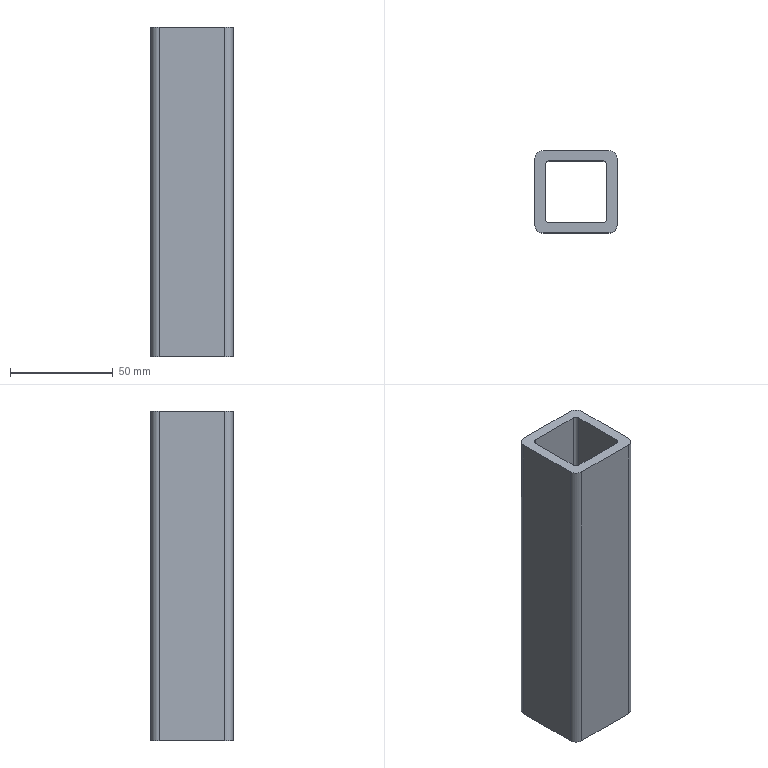Component | SolidWorks | 40-40SquareTube8-2 | 1 solid | 18 faces | box 40 x 40 x 160 mm | volume 110352 mm3 | plane 10 | cylinder 8 | commonest cylinder face diameters 8 x4 4 x4
build123d program:
from build123d import *

# Parameters (mm, degrees)
BOSS_EXTRUDE1_DEPTH = 80


with BuildPart() as part:
    # Sketch1 → Boss-Extrude1 (new, symmetric)
    with BuildSketch(Plane.XY):
        with BuildLine():
            Line((-16, -20), (16, -20))
            ThreePointArc((16, -20), (18.828, -18.828), (20, -16))
            Line((20, -16), (20, 16))
            ThreePointArc((20, 16), (18.828, 18.828), (16, 20))
            Line((16, 20), (-16, 20))
            ThreePointArc((-16, 20), (-18.828, 18.828), (-20, 16))
            Line((-20, 16), (-20, -16))
            ThreePointArc((-20, -16), (-18.828, -18.828), (-16, -20))
        make_face()
        with BuildLine():
            Line((-13, -15), (13, -15))
            ThreePointArc((13, -15), (14.414, -14.414), (15, -13))
            Line((15, -13), (15, 13))
            ThreePointArc((15, 13), (14.414, 14.414), (13, 15))
            Line((13, 15), (-13, 15))
            ThreePointArc((-13, 15), (-14.414, 14.414), (-15, 13))
            Line((-15, 13), (-15, -13))
            ThreePointArc((-15, -13), (-14.414, -14.414), (-13, -15))
        make_face(mode=Mode.SUBTRACT)
    extrude(amount=BOSS_EXTRUDE1_DEPTH, both=True)


solid = part.part

# Placed as in the assembly
solid = solid.moved(Location((17.398, 447.837, 100), (0, 0, 0)))
STEP:
#1=CARTESIAN_POINT('',(1.315,16.844,7.087));
#2=VERTEX_POINT('',#1);
#3=CARTESIAN_POINT('',(1.472,17.001,7.087));
#4=VERTEX_POINT('',#3);
#5=CARTESIAN_POINT('',(1.315,17.001,7.087));
#6=DIRECTION('',(0.,0.,1.));
#7=DIRECTION('',(1.,0.,0.));
#8=AXIS2_PLACEMENT_3D('',#5,#6,#7);
#9=CIRCLE('',#8,0.1575);
#10=EDGE_CURVE('',#2,#4,#9,.T.);
#11=ORIENTED_EDGE('',*,*,#10,.T.);
#12=CARTESIAN_POINT('',(1.472,18.261,7.087));
#13=VERTEX_POINT('',#12);
#14=CARTESIAN_POINT('',(1.472,17.001,7.087));
#15=DIRECTION('',(0.,1.,0.));
#16=VECTOR('',#15,39.37);
#17=LINE('',#14,#16);
#18=EDGE_CURVE('',#4,#13,#17,.T.);
#19=ORIENTED_EDGE('',*,*,#18,.T.);
#20=CARTESIAN_POINT('',(1.315,18.419,7.087));
#21=VERTEX_POINT('',#20);
#22=CARTESIAN_POINT('',(1.315,18.261,7.087));
#23=DIRECTION('',(0.,0.,1.));
#24=DIRECTION('',(-1.,0.,0.));
#25=AXIS2_PLACEMENT_3D('',#22,#23,#24);
#26=CIRCLE('',#25,0.1575);
#27=EDGE_CURVE('',#13,#21,#26,.T.);
#28=ORIENTED_EDGE('',*,*,#27,.T.);
#29=CARTESIAN_POINT('',(0.05504,18.419,7.087));
#30=VERTEX_POINT('',#29);
#31=CARTESIAN_POINT('',(0.05504,18.419,7.087));
#32=DIRECTION('',(-1.,0.,0.));
#33=VECTOR('',#32,39.37);
#34=LINE('',#31,#33);
#35=EDGE_CURVE('',#21,#30,#34,.T.);
#36=ORIENTED_EDGE('',*,*,#35,.T.);
#37=CARTESIAN_POINT('',(-0.1024,18.261,7.087));
#38=VERTEX_POINT('',#37);
#39=CARTESIAN_POINT('',(0.05504,18.261,7.087));
#40=DIRECTION('',(0.,0.,1.));
#41=DIRECTION('',(-1.,0.,0.));
#42=AXIS2_PLACEMENT_3D('',#39,#40,#41);
#43=CIRCLE('',#42,0.1575);
#44=EDGE_CURVE('',#30,#38,#43,.T.);
#45=ORIENTED_EDGE('',*,*,#44,.T.);
#46=CARTESIAN_POINT('',(-0.1024,17.001,7.087));
#47=VERTEX_POINT('',#46);
#48=CARTESIAN_POINT('',(-0.1024,17.001,7.087));
#49=DIRECTION('',(-0.,-1.,0.));
#50=VECTOR('',#49,39.37);
#51=LINE('',#48,#50);
#52=EDGE_CURVE('',#38,#47,#51,.T.);
#53=ORIENTED_EDGE('',*,*,#52,.T.);
#54=CARTESIAN_POINT('',(0.05504,16.844,7.087));
#55=VERTEX_POINT('',#54);
#56=CARTESIAN_POINT('',(0.05504,17.001,7.087));
#57=DIRECTION('',(0.,0.,1.));
#58=DIRECTION('',(-1.,0.,0.));
#59=AXIS2_PLACEMENT_3D('',#56,#57,#58);
#60=CIRCLE('',#59,0.1575);
#61=EDGE_CURVE('',#47,#55,#60,.T.);
#62=ORIENTED_EDGE('',*,*,#61,.T.);
#63=CARTESIAN_POINT('',(0.05504,16.844,7.087));
#64=DIRECTION('',(1.,0.,0.));
#65=VECTOR('',#64,39.37);
#66=LINE('',#63,#65);
#67=EDGE_CURVE('',#55,#2,#66,.T.);
#68=ORIENTED_EDGE('',*,*,#67,.T.);
#69=EDGE_LOOP('',(#11,#19,#28,#36,#45,#53,#62,#68));
#70=FACE_OUTER_BOUND('',#69,.T.);
#71=CARTESIAN_POINT('',(1.276,17.12,7.087));
#72=VERTEX_POINT('',#71);
#73=CARTESIAN_POINT('',(1.276,18.143,7.087));
#74=VERTEX_POINT('',#73);
#75=CARTESIAN_POINT('',(1.276,17.12,7.087));
#76=DIRECTION('',(0.,1.,0.));
#77=VECTOR('',#76,39.37);
#78=LINE('',#75,#77);
#79=EDGE_CURVE('',#72,#74,#78,.T.);
#80=ORIENTED_EDGE('',*,*,#79,.F.);
#81=CARTESIAN_POINT('',(1.197,17.041,7.087));
#82=VERTEX_POINT('',#81);
#83=CARTESIAN_POINT('',(1.197,17.12,7.087));
#84=DIRECTION('',(0.,0.,1.));
#85=DIRECTION('',(1.,0.,0.));
#86=AXIS2_PLACEMENT_3D('',#83,#84,#85);
#87=CIRCLE('',#86,0.07874);
#88=EDGE_CURVE('',#82,#72,#87,.T.);
#89=ORIENTED_EDGE('',*,*,#88,.F.);
#90=CARTESIAN_POINT('',(0.1732,17.041,7.087));
#91=VERTEX_POINT('',#90);
#92=CARTESIAN_POINT('',(0.1732,17.041,7.087));
#93=DIRECTION('',(1.,0.,0.));
#94=VECTOR('',#93,39.37);
#95=LINE('',#92,#94);
#96=EDGE_CURVE('',#91,#82,#95,.T.);
#97=ORIENTED_EDGE('',*,*,#96,.F.);
#98=CARTESIAN_POINT('',(0.09441,17.12,7.087));
#99=VERTEX_POINT('',#98);
#100=CARTESIAN_POINT('',(0.1732,17.12,7.087));
#101=DIRECTION('',(0.,0.,1.));
#102=DIRECTION('',(-1.,0.,0.));
#103=AXIS2_PLACEMENT_3D('',#100,#101,#102);
#104=CIRCLE('',#103,0.07874);
#105=EDGE_CURVE('',#99,#91,#104,.T.);
#106=ORIENTED_EDGE('',*,*,#105,.F.);
#107=CARTESIAN_POINT('',(0.09441,18.143,7.087));
#108=VERTEX_POINT('',#107);
#109=CARTESIAN_POINT('',(0.09441,17.12,7.087));
#110=DIRECTION('',(0.,-1.,0.));
#111=VECTOR('',#110,39.37);
#112=LINE('',#109,#111);
#113=EDGE_CURVE('',#108,#99,#112,.T.);
#114=ORIENTED_EDGE('',*,*,#113,.F.);
#115=CARTESIAN_POINT('',(0.1732,18.222,7.087));
#116=VERTEX_POINT('',#115);
#117=CARTESIAN_POINT('',(0.1732,18.143,7.087));
#118=DIRECTION('',(0.,0.,1.));
#119=DIRECTION('',(-1.,0.,0.));
#120=AXIS2_PLACEMENT_3D('',#117,#118,#119);
#121=CIRCLE('',#120,0.07874);
#122=EDGE_CURVE('',#116,#108,#121,.T.);
#123=ORIENTED_EDGE('',*,*,#122,.F.);
#124=CARTESIAN_POINT('',(1.197,18.222,7.087));
#125=VERTEX_POINT('',#124);
#126=CARTESIAN_POINT('',(0.1732,18.222,7.087));
#127=DIRECTION('',(-1.,0.,0.));
#128=VECTOR('',#127,39.37);
#129=LINE('',#126,#128);
#130=EDGE_CURVE('',#125,#116,#129,.T.);
#131=ORIENTED_EDGE('',*,*,#130,.F.);
#132=CARTESIAN_POINT('',(1.197,18.143,7.087));
#133=DIRECTION('',(0.,0.,1.));
#134=DIRECTION('',(-1.,0.,0.));
#135=AXIS2_PLACEMENT_3D('',#132,#133,#134);
#136=CIRCLE('',#135,0.07874);
#137=EDGE_CURVE('',#74,#125,#136,.T.);
#138=ORIENTED_EDGE('',*,*,#137,.F.);
#139=EDGE_LOOP('',(#80,#89,#97,#106,#114,#123,#131,#138));
#140=FACE_BOUND('',#139,.T.);
#141=CARTESIAN_POINT('',(1.315,17.001,7.087));
#142=DIRECTION('',(0.,0.,1.));
#143=DIRECTION('',(1.,0.,0.));
#144=AXIS2_PLACEMENT_3D('',#141,#142,#143);
#145=PLANE('',#144);
#146=ADVANCED_FACE('',(#70,#140),#145,.T.);
#147=CARTESIAN_POINT('',(1.315,16.844,0.7874));
#148=VERTEX_POINT('',#147);
#149=CARTESIAN_POINT('',(1.472,17.001,0.7874));
#150=VERTEX_POINT('',#149);
#151=CARTESIAN_POINT('',(1.315,17.001,0.7874));
#152=DIRECTION('',(0.,0.,1.));
#153=DIRECTION('',(1.,0.,0.));
#154=AXIS2_PLACEMENT_3D('',#151,#152,#153);
#155=CIRCLE('',#154,0.1575);
#156=EDGE_CURVE('',#148,#150,#155,.T.);
#157=ORIENTED_EDGE('',*,*,#156,.F.);
#158=CARTESIAN_POINT('',(0.05504,16.844,0.7874));
#159=VERTEX_POINT('',#158);
#160=CARTESIAN_POINT('',(0.05504,16.844,0.7874));
#161=DIRECTION('',(1.,0.,0.));
#162=VECTOR('',#161,39.37);
#163=LINE('',#160,#162);
#164=EDGE_CURVE('',#159,#148,#163,.T.);
#165=ORIENTED_EDGE('',*,*,#164,.F.);
#166=CARTESIAN_POINT('',(-0.1024,17.001,0.7874));
#167=VERTEX_POINT('',#166);
#168=CARTESIAN_POINT('',(0.05504,17.001,0.7874));
#169=DIRECTION('',(0.,0.,1.));
#170=DIRECTION('',(-1.,0.,0.));
#171=AXIS2_PLACEMENT_3D('',#168,#169,#170);
#172=CIRCLE('',#171,0.1575);
#173=EDGE_CURVE('',#167,#159,#172,.T.);
#174=ORIENTED_EDGE('',*,*,#173,.F.);
#175=CARTESIAN_POINT('',(-0.1024,18.261,0.7874));
#176=VERTEX_POINT('',#175);
#177=CARTESIAN_POINT('',(-0.1024,17.001,0.7874));
#178=DIRECTION('',(-0.,-1.,0.));
#179=VECTOR('',#178,39.37);
#180=LINE('',#177,#179);
#181=EDGE_CURVE('',#176,#167,#180,.T.);
#182=ORIENTED_EDGE('',*,*,#181,.F.);
#183=CARTESIAN_POINT('',(0.05504,18.419,0.7874));
#184=VERTEX_POINT('',#183);
#185=CARTESIAN_POINT('',(0.05504,18.261,0.7874));
#186=DIRECTION('',(0.,0.,1.));
#187=DIRECTION('',(-1.,0.,0.));
#188=AXIS2_PLACEMENT_3D('',#185,#186,#187);
#189=CIRCLE('',#188,0.1575);
#190=EDGE_CURVE('',#184,#176,#189,.T.);
#191=ORIENTED_EDGE('',*,*,#190,.F.);
#192=CARTESIAN_POINT('',(1.315,18.419,0.7874));
#193=VERTEX_POINT('',#192);
#194=CARTESIAN_POINT('',(0.05504,18.419,0.7874));
#195=DIRECTION('',(-1.,0.,0.));
#196=VECTOR('',#195,39.37);
#197=LINE('',#194,#196);
#198=EDGE_CURVE('',#193,#184,#197,.T.);
#199=ORIENTED_EDGE('',*,*,#198,.F.);
#200=CARTESIAN_POINT('',(1.472,18.261,0.7874));
#201=VERTEX_POINT('',#200);
#202=CARTESIAN_POINT('',(1.315,18.261,0.7874));
#203=DIRECTION('',(0.,0.,1.));
#204=DIRECTION('',(-1.,0.,0.));
#205=AXIS2_PLACEMENT_3D('',#202,#203,#204);
#206=CIRCLE('',#205,0.1575);
#207=EDGE_CURVE('',#201,#193,#206,.T.);
#208=ORIENTED_EDGE('',*,*,#207,.F.);
#209=CARTESIAN_POINT('',(1.472,17.001,0.7874));
#210=DIRECTION('',(0.,1.,0.));
#211=VECTOR('',#210,39.37);
#212=LINE('',#209,#211);
#213=EDGE_CURVE('',#150,#201,#212,.T.);
#214=ORIENTED_EDGE('',*,*,#213,.F.);
#215=EDGE_LOOP('',(#157,#165,#174,#182,#191,#199,#208,#214));
#216=FACE_OUTER_BOUND('',#215,.T.);
#217=CARTESIAN_POINT('',(1.197,17.041,0.7874));
#218=VERTEX_POINT('',#217);
#219=CARTESIAN_POINT('',(1.276,17.12,0.7874));
#220=VERTEX_POINT('',#219);
#221=CARTESIAN_POINT('',(1.197,17.12,0.7874));
#222=DIRECTION('',(0.,0.,1.));
#223=DIRECTION('',(1.,0.,0.));
#224=AXIS2_PLACEMENT_3D('',#221,#222,#223);
#225=CIRCLE('',#224,0.07874);
#226=EDGE_CURVE('',#218,#220,#225,.T.);
#227=ORIENTED_EDGE('',*,*,#226,.T.);
#228=CARTESIAN_POINT('',(1.276,18.143,0.7874));
#229=VERTEX_POINT('',#228);
#230=CARTESIAN_POINT('',(1.276,17.12,0.7874));
#231=DIRECTION('',(0.,1.,0.));
#232=VECTOR('',#231,39.37);
#233=LINE('',#230,#232);
#234=EDGE_CURVE('',#220,#229,#233,.T.);
#235=ORIENTED_EDGE('',*,*,#234,.T.);
#236=CARTESIAN_POINT('',(1.197,18.222,0.7874));
#237=VERTEX_POINT('',#236);
#238=CARTESIAN_POINT('',(1.197,18.143,0.7874));
#239=DIRECTION('',(0.,0.,1.));
#240=DIRECTION('',(-1.,0.,0.));
#241=AXIS2_PLACEMENT_3D('',#238,#239,#240);
#242=CIRCLE('',#241,0.07874);
#243=EDGE_CURVE('',#229,#237,#242,.T.);
#244=ORIENTED_EDGE('',*,*,#243,.T.);
#245=CARTESIAN_POINT('',(0.1732,18.222,0.7874));
#246=VERTEX_POINT('',#245);
#247=CARTESIAN_POINT('',(0.1732,18.222,0.7874));
#248=DIRECTION('',(-1.,0.,0.));
#249=VECTOR('',#248,39.37);
#250=LINE('',#247,#249);
#251=EDGE_CURVE('',#237,#246,#250,.T.);
#252=ORIENTED_EDGE('',*,*,#251,.T.);
#253=CARTESIAN_POINT('',(0.09441,18.143,0.7874));
#254=VERTEX_POINT('',#253);
#255=CARTESIAN_POINT('',(0.1732,18.143,0.7874));
#256=DIRECTION('',(0.,0.,1.));
#257=DIRECTION('',(-1.,0.,0.));
#258=AXIS2_PLACEMENT_3D('',#255,#256,#257);
#259=CIRCLE('',#258,0.07874);
#260=EDGE_CURVE('',#246,#254,#259,.T.);
#261=ORIENTED_EDGE('',*,*,#260,.T.);
#262=CARTESIAN_POINT('',(0.09441,17.12,0.7874));
#263=VERTEX_POINT('',#262);
#264=CARTESIAN_POINT('',(0.09441,17.12,0.7874));
#265=DIRECTION('',(0.,-1.,0.));
#266=VECTOR('',#265,39.37);
#267=LINE('',#264,#266);
#268=EDGE_CURVE('',#254,#263,#267,.T.);
#269=ORIENTED_EDGE('',*,*,#268,.T.);
#270=CARTESIAN_POINT('',(0.1732,17.041,0.7874));
#271=VERTEX_POINT('',#270);
#272=CARTESIAN_POINT('',(0.1732,17.12,0.7874));
#273=DIRECTION('',(0.,0.,1.));
#274=DIRECTION('',(-1.,0.,0.));
#275=AXIS2_PLACEMENT_3D('',#272,#273,#274);
#276=CIRCLE('',#275,0.07874);
#277=EDGE_CURVE('',#263,#271,#276,.T.);
#278=ORIENTED_EDGE('',*,*,#277,.T.);
#279=CARTESIAN_POINT('',(0.1732,17.041,0.7874));
#280=DIRECTION('',(1.,0.,0.));
#281=VECTOR('',#280,39.37);
#282=LINE('',#279,#281);
#283=EDGE_CURVE('',#271,#218,#282,.T.);
#284=ORIENTED_EDGE('',*,*,#283,.T.);
#285=EDGE_LOOP('',(#227,#235,#244,#252,#261,#269,#278,#284));
#286=FACE_BOUND('',#285,.T.);
#287=CARTESIAN_POINT('',(1.315,17.001,0.7874));
#288=DIRECTION('',(0.,0.,1.));
#289=DIRECTION('',(1.,0.,0.));
#290=AXIS2_PLACEMENT_3D('',#287,#288,#289);
#291=PLANE('',#290);
#292=ADVANCED_FACE('',(#216,#286),#291,.F.);
#293=ORIENTED_EDGE('',*,*,#156,.T.);
#294=CARTESIAN_POINT('',(1.472,17.001,7.087));
#295=DIRECTION('',(0.,0.,-1.));
#296=VECTOR('',#295,39.37);
#297=LINE('',#294,#296);
#298=EDGE_CURVE('',#4,#150,#297,.T.);
#299=ORIENTED_EDGE('',*,*,#298,.F.);
#300=ORIENTED_EDGE('',*,*,#10,.F.);
#301=CARTESIAN_POINT('',(1.315,16.844,7.087));
#302=DIRECTION('',(0.,0.,-1.));
#303=VECTOR('',#302,39.37);
#304=LINE('',#301,#303);
#305=EDGE_CURVE('',#2,#148,#304,.T.);
#306=ORIENTED_EDGE('',*,*,#305,.T.);
#307=EDGE_LOOP('',(#293,#299,#300,#306));
#308=FACE_OUTER_BOUND('',#307,.T.);
#309=CARTESIAN_POINT('',(1.315,17.001,7.087));
#310=DIRECTION('',(0.,0.,-1.));
#311=DIRECTION('',(-1.,0.,0.));
#312=AXIS2_PLACEMENT_3D('',#309,#310,#311);
#313=CYLINDRICAL_SURFACE('',#312,0.1575);
#314=ADVANCED_FACE('',(#308),#313,.T.);
#315=ORIENTED_EDGE('',*,*,#213,.T.);
#316=CARTESIAN_POINT('',(1.472,18.261,7.087));
#317=DIRECTION('',(0.,0.,-1.));
#318=VECTOR('',#317,39.37);
#319=LINE('',#316,#318);
#320=EDGE_CURVE('',#13,#201,#319,.T.);
#321=ORIENTED_EDGE('',*,*,#320,.F.);
#322=ORIENTED_EDGE('',*,*,#18,.F.);
#323=ORIENTED_EDGE('',*,*,#298,.T.);
#324=EDGE_LOOP('',(#315,#321,#322,#323));
#325=FACE_OUTER_BOUND('',#324,.T.);
#326=CARTESIAN_POINT('',(1.472,17.001,7.087));
#327=DIRECTION('',(-1.,0.,0.));
#328=DIRECTION('',(0.,0.,1.));
#329=AXIS2_PLACEMENT_3D('',#326,#327,#328);
#330=PLANE('',#329);
#331=ADVANCED_FACE('',(#325),#330,.F.);
#332=ORIENTED_EDGE('',*,*,#207,.T.);
#333=CARTESIAN_POINT('',(1.315,18.419,7.087));
#334=DIRECTION('',(0.,0.,-1.));
#335=VECTOR('',#334,39.37);
#336=LINE('',#333,#335);
#337=EDGE_CURVE('',#21,#193,#336,.T.);
#338=ORIENTED_EDGE('',*,*,#337,.F.);
#339=ORIENTED_EDGE('',*,*,#27,.F.);
#340=ORIENTED_EDGE('',*,*,#320,.T.);
#341=EDGE_LOOP('',(#332,#338,#339,#340));
#342=FACE_OUTER_BOUND('',#341,.T.);
#343=CARTESIAN_POINT('',(1.315,18.261,7.087));
#344=DIRECTION('',(0.,0.,-1.));
#345=DIRECTION('',(-1.,0.,0.));
#346=AXIS2_PLACEMENT_3D('',#343,#344,#345);
#347=CYLINDRICAL_SURFACE('',#346,0.1575);
#348=ADVANCED_FACE('',(#342),#347,.T.);
#349=ORIENTED_EDGE('',*,*,#198,.T.);
#350=CARTESIAN_POINT('',(0.05504,18.419,7.087));
#351=DIRECTION('',(0.,0.,-1.));
#352=VECTOR('',#351,39.37);
#353=LINE('',#350,#352);
#354=EDGE_CURVE('',#30,#184,#353,.T.);
#355=ORIENTED_EDGE('',*,*,#354,.F.);
#356=ORIENTED_EDGE('',*,*,#35,.F.);
#357=ORIENTED_EDGE('',*,*,#337,.T.);
#358=EDGE_LOOP('',(#349,#355,#356,#357));
#359=FACE_OUTER_BOUND('',#358,.T.);
#360=CARTESIAN_POINT('',(0.05504,18.419,7.087));
#361=DIRECTION('',(0.,-1.,0.));
#362=DIRECTION('',(0.,0.,-1.));
#363=AXIS2_PLACEMENT_3D('',#360,#361,#362);
#364=PLANE('',#363);
#365=ADVANCED_FACE('',(#359),#364,.F.);
#366=ORIENTED_EDGE('',*,*,#190,.T.);
#367=CARTESIAN_POINT('',(-0.1024,18.261,7.087));
#368=DIRECTION('',(0.,0.,-1.));
#369=VECTOR('',#368,39.37);
#370=LINE('',#367,#369);
#371=EDGE_CURVE('',#38,#176,#370,.T.);
#372=ORIENTED_EDGE('',*,*,#371,.F.);
#373=ORIENTED_EDGE('',*,*,#44,.F.);
#374=ORIENTED_EDGE('',*,*,#354,.T.);
#375=EDGE_LOOP('',(#366,#372,#373,#374));
#376=FACE_OUTER_BOUND('',#375,.T.);
#377=CARTESIAN_POINT('',(0.05504,18.261,7.087));
#378=DIRECTION('',(0.,0.,-1.));
#379=DIRECTION('',(-1.,0.,0.));
#380=AXIS2_PLACEMENT_3D('',#377,#378,#379);
#381=CYLINDRICAL_SURFACE('',#380,0.1575);
#382=ADVANCED_FACE('',(#376),#381,.T.);
#383=ORIENTED_EDGE('',*,*,#181,.T.);
#384=CARTESIAN_POINT('',(-0.1024,17.001,7.087));
#385=DIRECTION('',(0.,0.,-1.));
#386=VECTOR('',#385,39.37);
#387=LINE('',#384,#386);
#388=EDGE_CURVE('',#47,#167,#387,.T.);
#389=ORIENTED_EDGE('',*,*,#388,.F.);
#390=ORIENTED_EDGE('',*,*,#52,.F.);
#391=ORIENTED_EDGE('',*,*,#371,.T.);
#392=EDGE_LOOP('',(#383,#389,#390,#391));
#393=FACE_OUTER_BOUND('',#392,.T.);
#394=CARTESIAN_POINT('',(-0.1024,17.001,7.087));
#395=DIRECTION('',(1.,-0.,0.));
#396=DIRECTION('',(0.,1.,0.));
#397=AXIS2_PLACEMENT_3D('',#394,#395,#396);
#398=PLANE('',#397);
#399=ADVANCED_FACE('',(#393),#398,.F.);
#400=ORIENTED_EDGE('',*,*,#173,.T.);
#401=CARTESIAN_POINT('',(0.05504,16.844,7.087));
#402=DIRECTION('',(0.,0.,-1.));
#403=VECTOR('',#402,39.37);
#404=LINE('',#401,#403);
#405=EDGE_CURVE('',#55,#159,#404,.T.);
#406=ORIENTED_EDGE('',*,*,#405,.F.);
#407=ORIENTED_EDGE('',*,*,#61,.F.);
#408=ORIENTED_EDGE('',*,*,#388,.T.);
#409=EDGE_LOOP('',(#400,#406,#407,#408));
#410=FACE_OUTER_BOUND('',#409,.T.);
#411=CARTESIAN_POINT('',(0.05504,17.001,7.087));
#412=DIRECTION('',(0.,0.,-1.));
#413=DIRECTION('',(-1.,0.,0.));
#414=AXIS2_PLACEMENT_3D('',#411,#412,#413);
#415=CYLINDRICAL_SURFACE('',#414,0.1575);
#416=ADVANCED_FACE('',(#410),#415,.T.);
#417=ORIENTED_EDGE('',*,*,#164,.T.);
#418=ORIENTED_EDGE('',*,*,#305,.F.);
#419=ORIENTED_EDGE('',*,*,#67,.F.);
#420=ORIENTED_EDGE('',*,*,#405,.T.);
#421=EDGE_LOOP('',(#417,#418,#419,#420));
#422=FACE_OUTER_BOUND('',#421,.T.);
#423=CARTESIAN_POINT('',(0.05504,16.844,7.087));
#424=DIRECTION('',(0.,1.,0.));
#425=DIRECTION('',(0.,0.,1.));
#426=AXIS2_PLACEMENT_3D('',#423,#424,#425);
#427=PLANE('',#426);
#428=ADVANCED_FACE('',(#422),#427,.F.);
#429=ORIENTED_EDGE('',*,*,#226,.F.);
#430=CARTESIAN_POINT('',(1.197,17.041,7.087));
#431=DIRECTION('',(0.,0.,-1.));
#432=VECTOR('',#431,39.37);
#433=LINE('',#430,#432);
#434=EDGE_CURVE('',#82,#218,#433,.T.);
#435=ORIENTED_EDGE('',*,*,#434,.F.);
#436=ORIENTED_EDGE('',*,*,#88,.T.);
#437=CARTESIAN_POINT('',(1.276,17.12,7.087));
#438=DIRECTION('',(0.,0.,-1.));
#439=VECTOR('',#438,39.37);
#440=LINE('',#437,#439);
#441=EDGE_CURVE('',#72,#220,#440,.T.);
#442=ORIENTED_EDGE('',*,*,#441,.T.);
#443=EDGE_LOOP('',(#429,#435,#436,#442));
#444=FACE_OUTER_BOUND('',#443,.T.);
#445=CARTESIAN_POINT('',(1.197,17.12,7.087));
#446=DIRECTION('',(0.,0.,-1.));
#447=DIRECTION('',(-1.,0.,0.));
#448=AXIS2_PLACEMENT_3D('',#445,#446,#447);
#449=CYLINDRICAL_SURFACE('',#448,0.07874);
#450=ADVANCED_FACE('',(#444),#449,.F.);
#451=ORIENTED_EDGE('',*,*,#234,.F.);
#452=ORIENTED_EDGE('',*,*,#441,.F.);
#453=ORIENTED_EDGE('',*,*,#79,.T.);
#454=CARTESIAN_POINT('',(1.276,18.143,7.087));
#455=DIRECTION('',(0.,0.,-1.));
#456=VECTOR('',#455,39.37);
#457=LINE('',#454,#456);
#458=EDGE_CURVE('',#74,#229,#457,.T.);
#459=ORIENTED_EDGE('',*,*,#458,.T.);
#460=EDGE_LOOP('',(#451,#452,#453,#459));
#461=FACE_OUTER_BOUND('',#460,.T.);
#462=CARTESIAN_POINT('',(1.276,17.12,7.087));
#463=DIRECTION('',(-1.,0.,0.));
#464=DIRECTION('',(0.,0.,1.));
#465=AXIS2_PLACEMENT_3D('',#462,#463,#464);
#466=PLANE('',#465);
#467=ADVANCED_FACE('',(#461),#466,.T.);
#468=ORIENTED_EDGE('',*,*,#243,.F.);
#469=ORIENTED_EDGE('',*,*,#458,.F.);
#470=ORIENTED_EDGE('',*,*,#137,.T.);
#471=CARTESIAN_POINT('',(1.197,18.222,7.087));
#472=DIRECTION('',(0.,0.,-1.));
#473=VECTOR('',#472,39.37);
#474=LINE('',#471,#473);
#475=EDGE_CURVE('',#125,#237,#474,.T.);
#476=ORIENTED_EDGE('',*,*,#475,.T.);
#477=EDGE_LOOP('',(#468,#469,#470,#476));
#478=FACE_OUTER_BOUND('',#477,.T.);
#479=CARTESIAN_POINT('',(1.197,18.143,7.087));
#480=DIRECTION('',(0.,0.,-1.));
#481=DIRECTION('',(-1.,0.,0.));
#482=AXIS2_PLACEMENT_3D('',#479,#480,#481);
#483=CYLINDRICAL_SURFACE('',#482,0.07874);
#484=ADVANCED_FACE('',(#478),#483,.F.);
#485=ORIENTED_EDGE('',*,*,#251,.F.);
#486=ORIENTED_EDGE('',*,*,#475,.F.);
#487=ORIENTED_EDGE('',*,*,#130,.T.);
#488=CARTESIAN_POINT('',(0.1732,18.222,7.087));
#489=DIRECTION('',(0.,0.,-1.));
#490=VECTOR('',#489,39.37);
#491=LINE('',#488,#490);
#492=EDGE_CURVE('',#116,#246,#491,.T.);
#493=ORIENTED_EDGE('',*,*,#492,.T.);
#494=EDGE_LOOP('',(#485,#486,#487,#493));
#495=FACE_OUTER_BOUND('',#494,.T.);
#496=CARTESIAN_POINT('',(0.1732,18.222,7.087));
#497=DIRECTION('',(0.,-1.,0.));
#498=DIRECTION('',(0.,0.,-1.));
#499=AXIS2_PLACEMENT_3D('',#496,#497,#498);
#500=PLANE('',#499);
#501=ADVANCED_FACE('',(#495),#500,.T.);
#502=ORIENTED_EDGE('',*,*,#260,.F.);
#503=ORIENTED_EDGE('',*,*,#492,.F.);
#504=ORIENTED_EDGE('',*,*,#122,.T.);
#505=CARTESIAN_POINT('',(0.09441,18.143,7.087));
#506=DIRECTION('',(0.,0.,-1.));
#507=VECTOR('',#506,39.37);
#508=LINE('',#505,#507);
#509=EDGE_CURVE('',#108,#254,#508,.T.);
#510=ORIENTED_EDGE('',*,*,#509,.T.);
#511=EDGE_LOOP('',(#502,#503,#504,#510));
#512=FACE_OUTER_BOUND('',#511,.T.);
#513=CARTESIAN_POINT('',(0.1732,18.143,7.087));
#514=DIRECTION('',(0.,0.,-1.));
#515=DIRECTION('',(-1.,0.,0.));
#516=AXIS2_PLACEMENT_3D('',#513,#514,#515);
#517=CYLINDRICAL_SURFACE('',#516,0.07874);
#518=ADVANCED_FACE('',(#512),#517,.F.);
#519=ORIENTED_EDGE('',*,*,#268,.F.);
#520=ORIENTED_EDGE('',*,*,#509,.F.);
#521=ORIENTED_EDGE('',*,*,#113,.T.);
#522=CARTESIAN_POINT('',(0.09441,17.12,7.087));
#523=DIRECTION('',(0.,0.,-1.));
#524=VECTOR('',#523,39.37);
#525=LINE('',#522,#524);
#526=EDGE_CURVE('',#99,#263,#525,.T.);
#527=ORIENTED_EDGE('',*,*,#526,.T.);
#528=EDGE_LOOP('',(#519,#520,#521,#527));
#529=FACE_OUTER_BOUND('',#528,.T.);
#530=CARTESIAN_POINT('',(0.09441,17.12,7.087));
#531=DIRECTION('',(1.,0.,0.));
#532=DIRECTION('',(0.,0.,-1.));
#533=AXIS2_PLACEMENT_3D('',#530,#531,#532);
#534=PLANE('',#533);
#535=ADVANCED_FACE('',(#529),#534,.T.);
#536=ORIENTED_EDGE('',*,*,#277,.F.);
#537=ORIENTED_EDGE('',*,*,#526,.F.);
#538=ORIENTED_EDGE('',*,*,#105,.T.);
#539=CARTESIAN_POINT('',(0.1732,17.041,7.087));
#540=DIRECTION('',(0.,0.,-1.));
#541=VECTOR('',#540,39.37);
#542=LINE('',#539,#541);
#543=EDGE_CURVE('',#91,#271,#542,.T.);
#544=ORIENTED_EDGE('',*,*,#543,.T.);
#545=EDGE_LOOP('',(#536,#537,#538,#544));
#546=FACE_OUTER_BOUND('',#545,.T.);
#547=CARTESIAN_POINT('',(0.1732,17.12,7.087));
#548=DIRECTION('',(0.,0.,-1.));
#549=DIRECTION('',(-1.,0.,0.));
#550=AXIS2_PLACEMENT_3D('',#547,#548,#549);
#551=CYLINDRICAL_SURFACE('',#550,0.07874);
#552=ADVANCED_FACE('',(#546),#551,.F.);
#553=ORIENTED_EDGE('',*,*,#283,.F.);
#554=ORIENTED_EDGE('',*,*,#543,.F.);
#555=ORIENTED_EDGE('',*,*,#96,.T.);
#556=ORIENTED_EDGE('',*,*,#434,.T.);
#557=EDGE_LOOP('',(#553,#554,#555,#556));
#558=FACE_OUTER_BOUND('',#557,.T.);
#559=CARTESIAN_POINT('',(0.1732,17.041,7.087));
#560=DIRECTION('',(0.,1.,0.));
#561=DIRECTION('',(0.,0.,1.));
#562=AXIS2_PLACEMENT_3D('',#559,#560,#561);
#563=PLANE('',#562);
#564=ADVANCED_FACE('',(#558),#563,.T.);
#565=CLOSED_SHELL('',(#146,#292,#314,#331,#348,#365,#382,#399,#416,#428,#450,#467,#484,#501,#518,#535,#552,#564));
#566=MANIFOLD_SOLID_BREP('',#565);
#567=CARTESIAN_POINT('',(0.,0.,0.));
#568=DIRECTION('',(0.,0.,1.));
#569=DIRECTION('',(1.,0.,0.));
#570=AXIS2_PLACEMENT_3D('',#567,#568,#569);
#571=(LENGTH_UNIT()NAMED_UNIT(*)SI_UNIT($,.METRE.));
#572=LENGTH_MEASURE_WITH_UNIT(LENGTH_MEASURE(0.0254),#571);
#573=DIMENSIONAL_EXPONENTS(1.,0.,0.,0.,0.,0.,0.);
#574=(CONVERSION_BASED_UNIT('',#572)LENGTH_UNIT()NAMED_UNIT(#573));
#575=UNCERTAINTY_MEASURE_WITH_UNIT(LENGTH_MEASURE(0.00001),#574,'','');
#576=(NAMED_UNIT(*)PLANE_ANGLE_UNIT()SI_UNIT($,.RADIAN.));
#577=(NAMED_UNIT(*)SI_UNIT($,.STERADIAN.)SOLID_ANGLE_UNIT());
#578=(GEOMETRIC_REPRESENTATION_CONTEXT(3)GLOBAL_UNCERTAINTY_ASSIGNED_CONTEXT((#575))GLOBAL_UNIT_ASSIGNED_CONTEXT((#574,#576,#577))REPRESENTATION_CONTEXT('',''));
#579=ADVANCED_BREP_SHAPE_REPRESENTATION('',(#566,#570),#578);
#580=COLOUR_RGB('',0.7922,0.8196,0.9333);
#581=FILL_AREA_STYLE_COLOUR('',#580);
#582=FILL_AREA_STYLE('',(#581));
#583=SURFACE_STYLE_FILL_AREA(#582);
#584=SURFACE_SIDE_STYLE('',(#583));
#585=SURFACE_STYLE_USAGE(.BOTH.,#584);
#586=PRESENTATION_STYLE_ASSIGNMENT((#585));
#587=STYLED_ITEM('',(#586),#566);
#588=(LENGTH_UNIT()NAMED_UNIT(*)SI_UNIT($,.METRE.));
#589=LENGTH_MEASURE_WITH_UNIT(LENGTH_MEASURE(0.0254),#588);
#590=DIMENSIONAL_EXPONENTS(1.,0.,0.,0.,0.,0.,0.);
#591=(CONVERSION_BASED_UNIT('',#589)LENGTH_UNIT()NAMED_UNIT(#590));
#592=UNCERTAINTY_MEASURE_WITH_UNIT(LENGTH_MEASURE(0.00001),#591,'','');
#593=(NAMED_UNIT(*)PLANE_ANGLE_UNIT()SI_UNIT($,.RADIAN.));
#594=(NAMED_UNIT(*)SI_UNIT($,.STERADIAN.)SOLID_ANGLE_UNIT());
#595=(GEOMETRIC_REPRESENTATION_CONTEXT(3)GLOBAL_UNCERTAINTY_ASSIGNED_CONTEXT((#592))GLOBAL_UNIT_ASSIGNED_CONTEXT((#591,#593,#594))REPRESENTATION_CONTEXT('',''));
#596=MECHANICAL_DESIGN_GEOMETRIC_PRESENTATION_REPRESENTATION('',(#587),#595);
#597=PRESENTATION_LAYER_ASSIGNMENT('','',(#587));